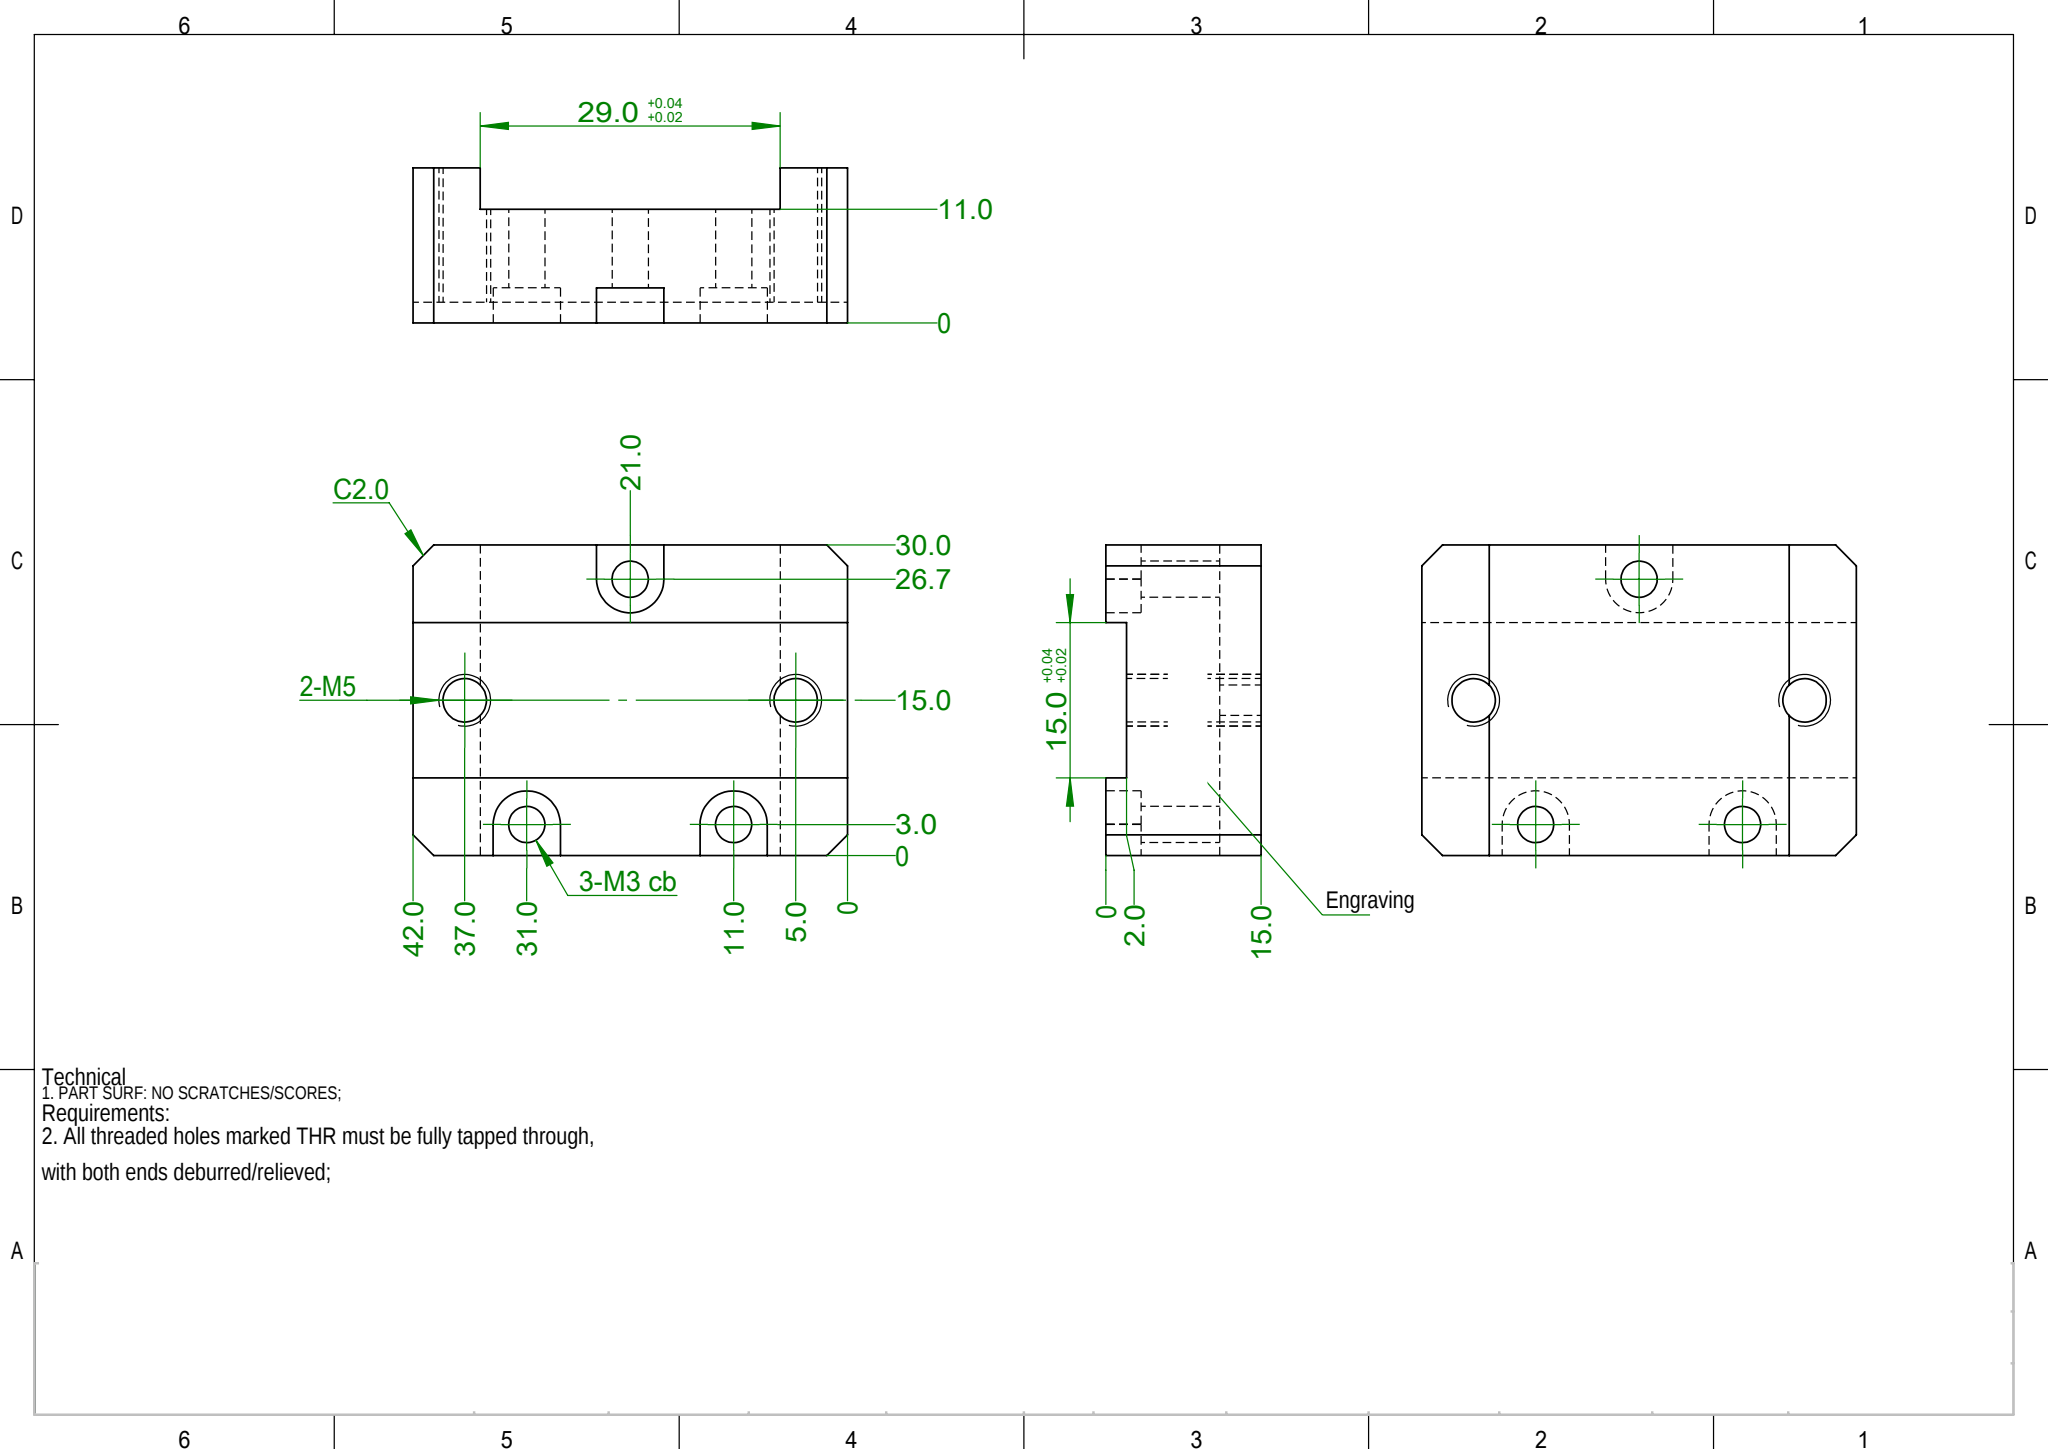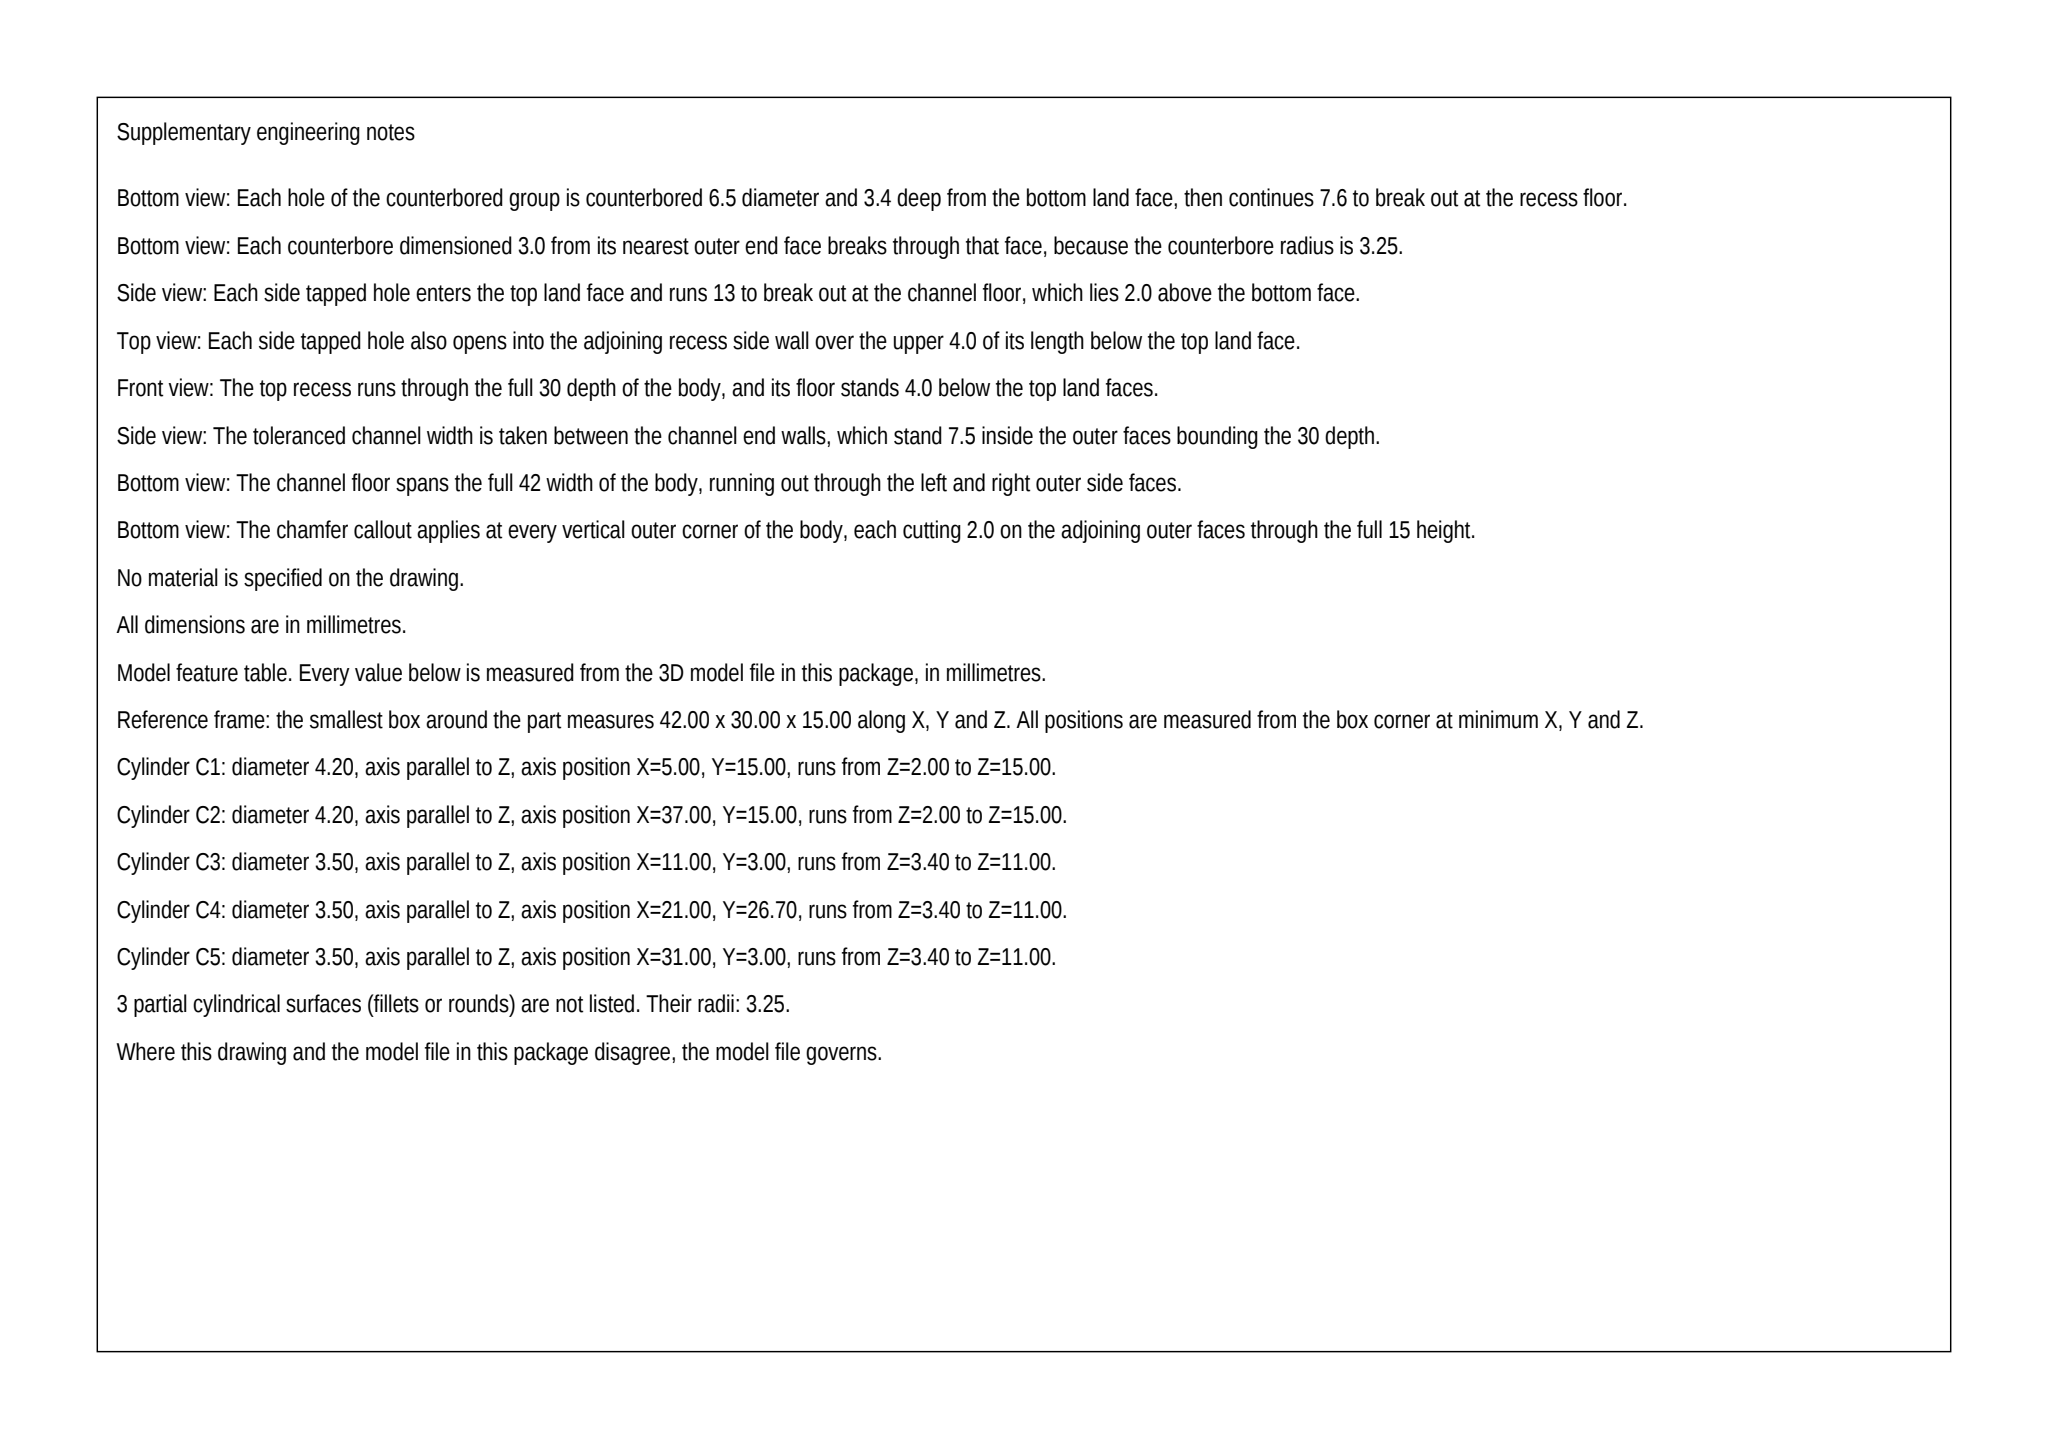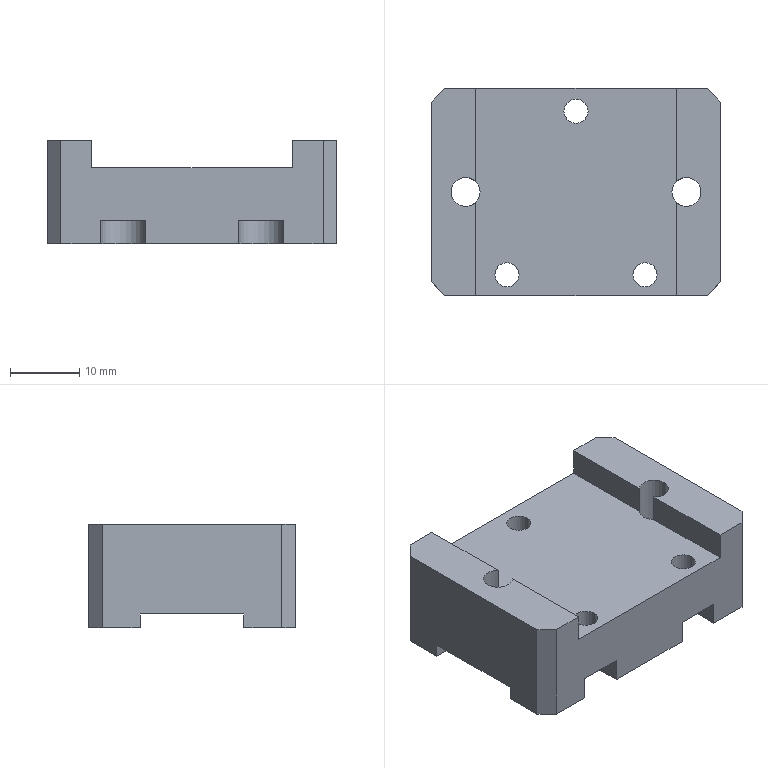Part | SolidWorks | mm | 1 solid | 42 faces | box 42 x 30 x 15 mm | volume 13095 mm3 | plane 29 | cylinder 13 | commonest cylinder face diameters 3.5 x6 4.2 x4 6.5 x3
Drawing notes:
3-M3 cb: C'BORE Ø6.5 | from the solid: cylinders dia 6.5 at (11,3),(21,26.7),(31,3), len 3.4
3-M3 cb: C'BORE DP 3.4 FROM BOTTOM FACE (Z0) | from the solid: Ø6.5 cyls run Z0 to Z3.4; z-planes at 0 and 3.4
UNLESS OTHERWISE SPECIFIED ALL DIMS IN MM | from the solid: STEP model units mm; bbox 42.0 x 30.0 x 15.0 mm